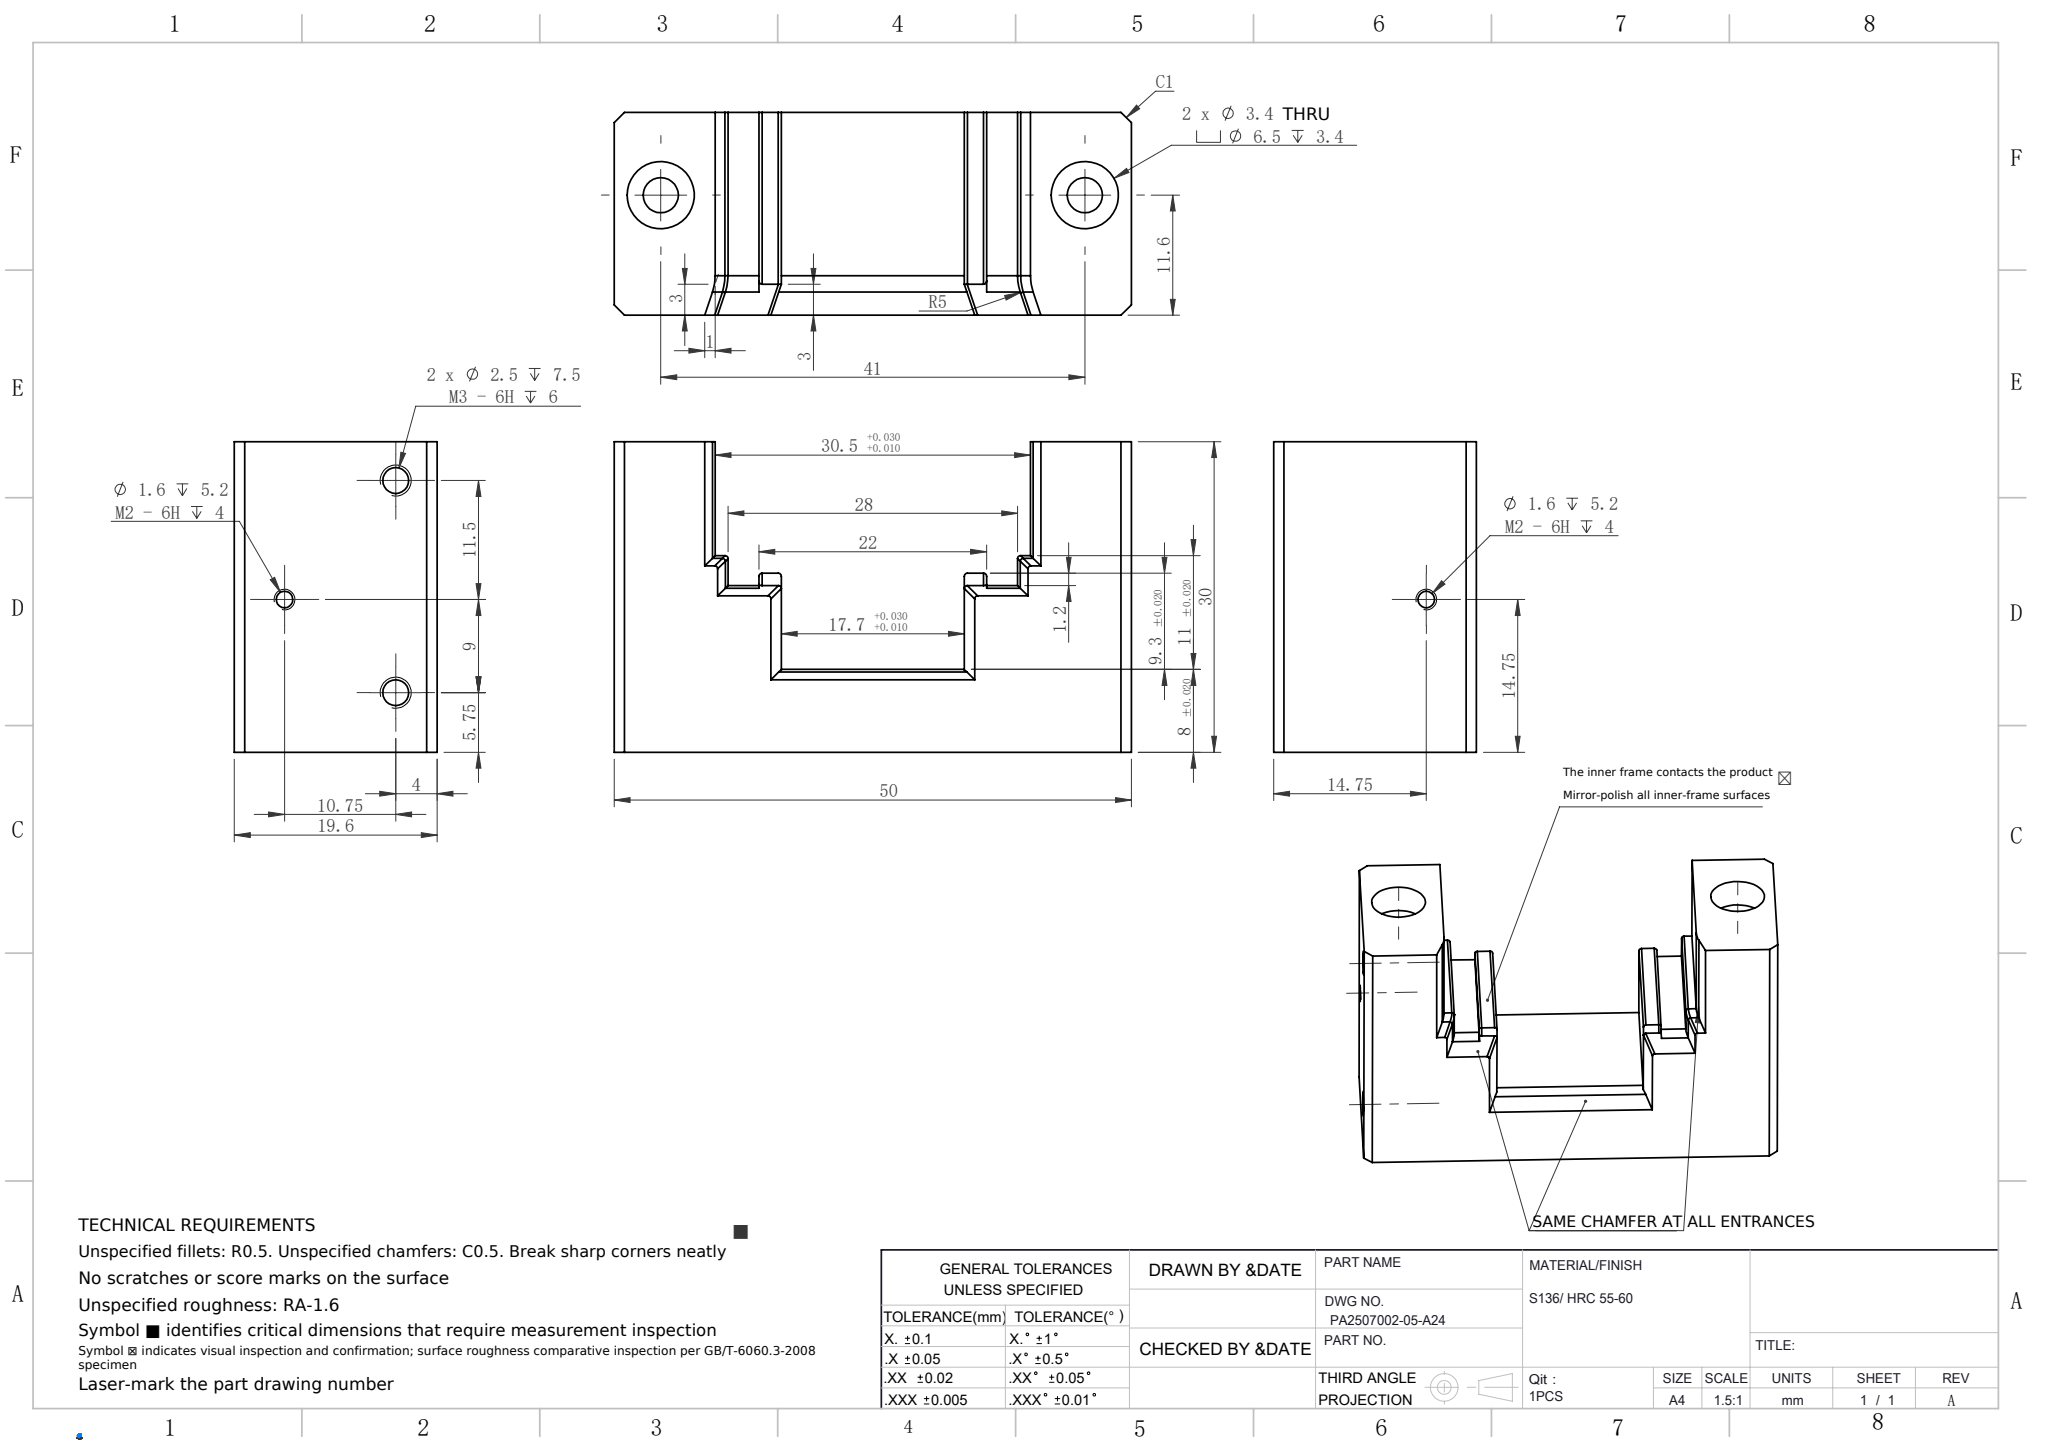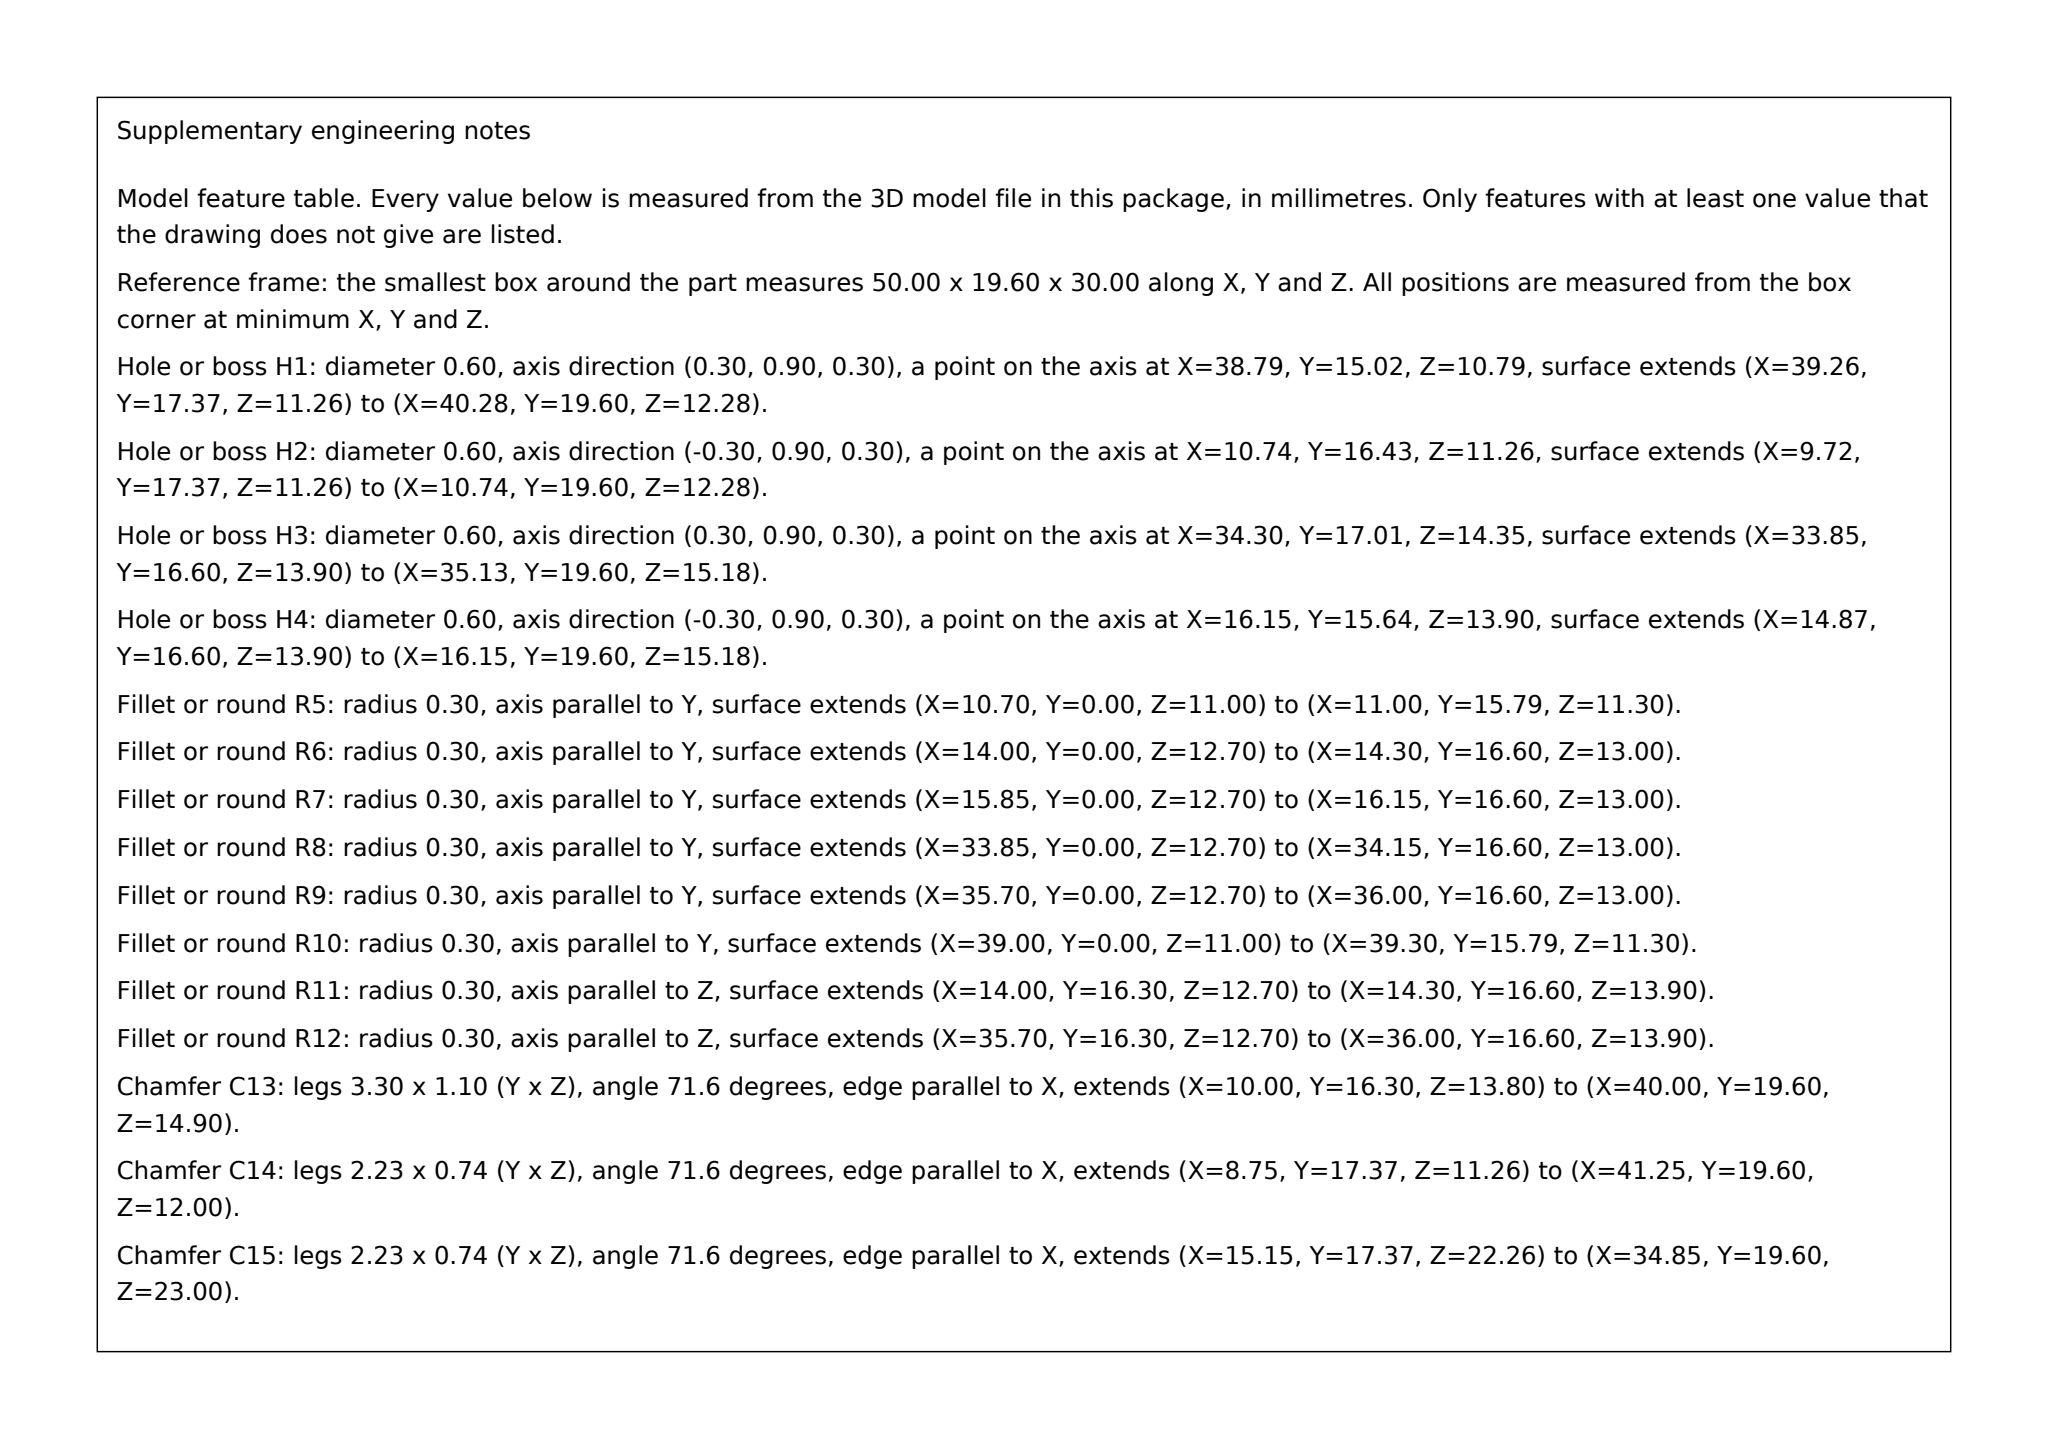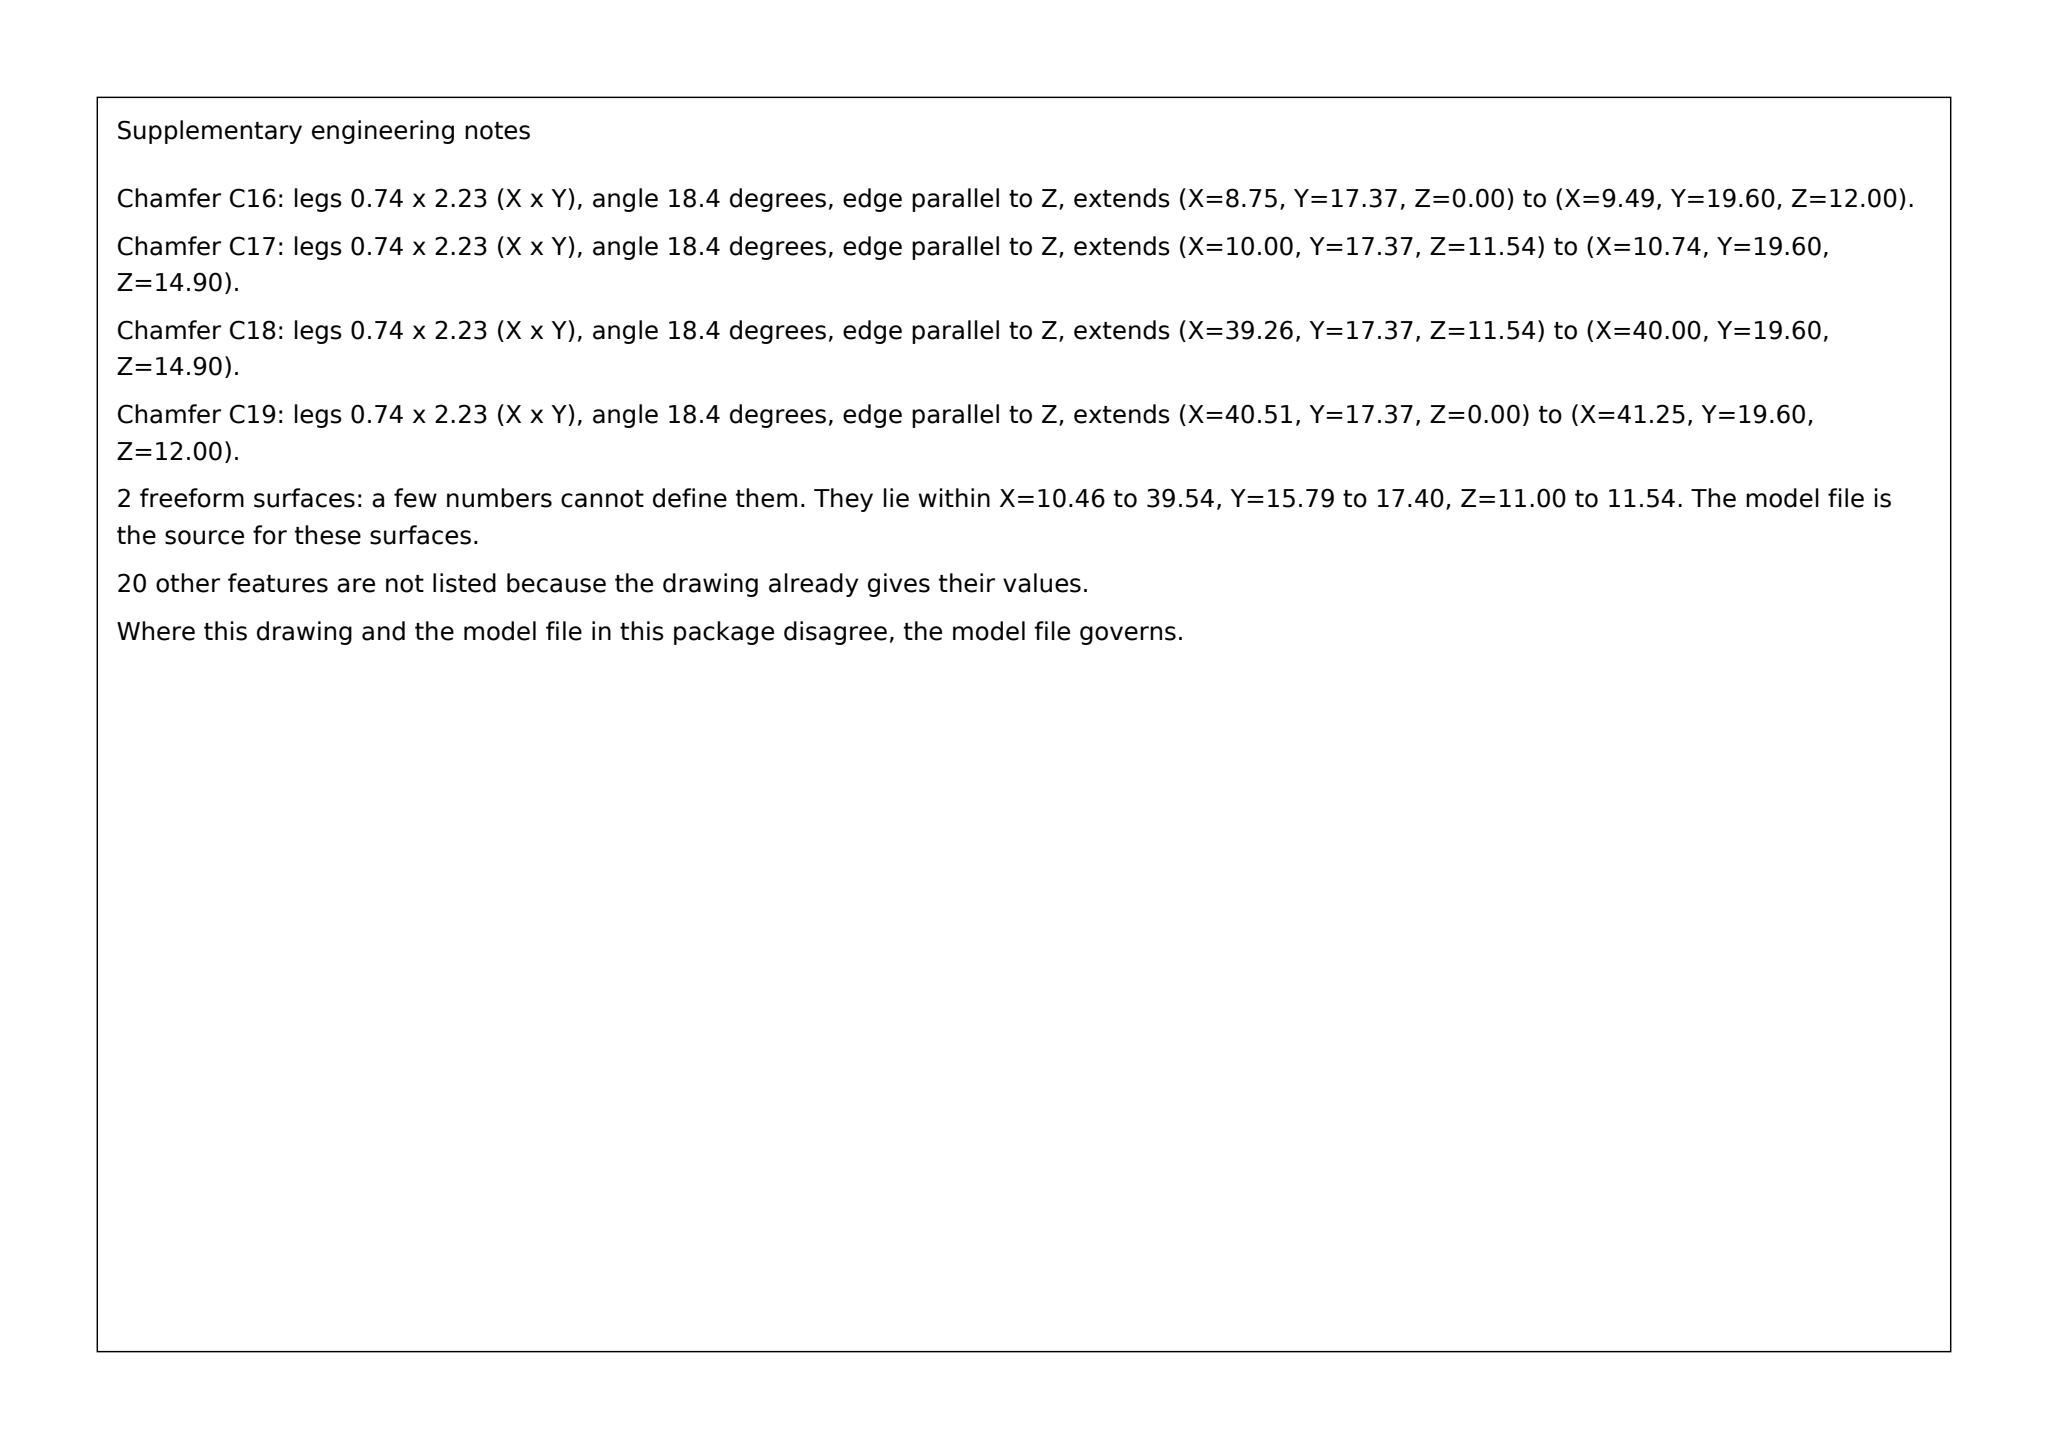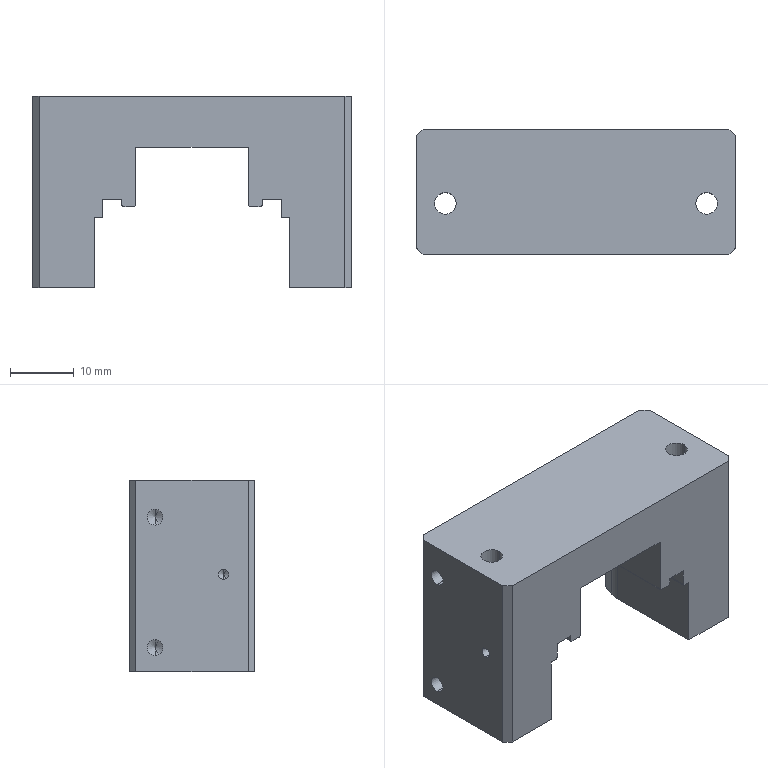Part | SolidWorks | mm | material S136/ HRC 55-60 | 1 solid | 88 faces | box 50 x 19.6 x 30 mm | volume 17524 mm3 | plane 41 | cylinder 37 | cone 8 | spline 2 | commonest cylinder face diameters 0.6 x12 10 x9 2.5 x4 1.6 x4 6.5 x4 3.4 x4